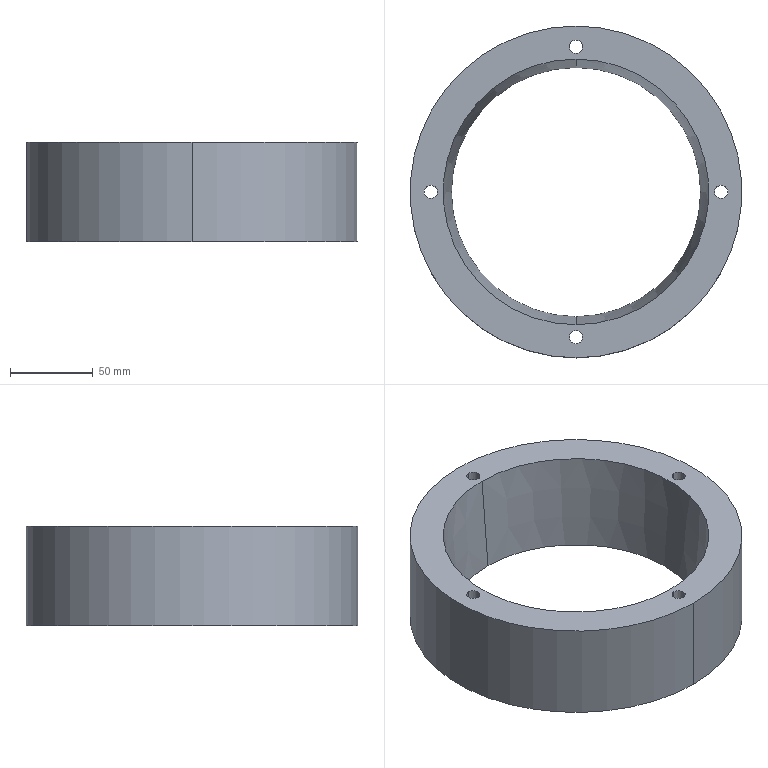Component | SolidWorks | DieStressRing-1 | 1 solid | 26 faces | box 200 x 200 x 60 mm | volume 718694 mm3 | cylinder 18 | plane 6 | cone 2 | commonest cylinder face diameters 16.5 x8 8 x8 200 x2
STEP:
#1=COLOUR_RGB('',0.7922,0.8196,0.9333);
#2=FILL_AREA_STYLE_COLOUR('',#1);
#3=FILL_AREA_STYLE('',(#2));
#4=SURFACE_STYLE_FILL_AREA(#3);
#5=SURFACE_SIDE_STYLE('',(#4));
#6=SURFACE_STYLE_USAGE(.BOTH.,#5);
#7=PRESENTATION_STYLE_ASSIGNMENT((#6));
#8=CARTESIAN_POINT('',(0.,-3.77,-3.071));
#9=VERTEX_POINT('',#8);
#10=CARTESIAN_POINT('',(0.,-3.12,-3.071));
#11=VERTEX_POINT('',#10);
#12=CARTESIAN_POINT('',(0.,-3.445,-3.071));
#13=DIRECTION('',(0.,0.,-1.));
#14=DIRECTION('',(-0.,1.,0.));
#15=AXIS2_PLACEMENT_3D('',#12,#13,#14);
#16=CIRCLE('',#15,0.3248);
#17=EDGE_CURVE('',#9,#11,#16,.T.);
#18=ORIENTED_EDGE('',*,*,#17,.F.);
#19=CARTESIAN_POINT('',(0.,-3.77,-4.252));
#20=VERTEX_POINT('',#19);
#21=CARTESIAN_POINT('',(0.,-3.77,-3.071));
#22=DIRECTION('',(0.,0.,-1.));
#23=VECTOR('',#22,39.37);
#24=LINE('',#21,#23);
#25=EDGE_CURVE('',#9,#20,#24,.T.);
#26=ORIENTED_EDGE('',*,*,#25,.T.);
#27=CARTESIAN_POINT('',(0.,-3.12,-4.252));
#28=VERTEX_POINT('',#27);
#29=CARTESIAN_POINT('',(0.,-3.445,-4.252));
#30=DIRECTION('',(0.,0.,-1.));
#31=DIRECTION('',(-0.,1.,0.));
#32=AXIS2_PLACEMENT_3D('',#29,#30,#31);
#33=CIRCLE('',#32,0.3248);
#34=EDGE_CURVE('',#20,#28,#33,.T.);
#35=ORIENTED_EDGE('',*,*,#34,.T.);
#36=CARTESIAN_POINT('',(0.,-3.12,-3.071));
#37=DIRECTION('',(0.,0.,-1.));
#38=VECTOR('',#37,39.37);
#39=LINE('',#36,#38);
#40=EDGE_CURVE('',#11,#28,#39,.T.);
#41=ORIENTED_EDGE('',*,*,#40,.F.);
#42=EDGE_LOOP('',(#18,#26,#35,#41));
#43=FACE_OUTER_BOUND('',#42,.T.);
#44=CARTESIAN_POINT('',(0.,-3.445,-3.071));
#45=DIRECTION('',(0.,0.,-1.));
#46=DIRECTION('',(-0.,1.,0.));
#47=AXIS2_PLACEMENT_3D('',#44,#45,#46);
#48=CYLINDRICAL_SURFACE('',#47,0.3248);
#49=ADVANCED_FACE('',(#43),#48,.F.);
#50=CARTESIAN_POINT('',(3.445,-0.3248,-3.071));
#51=VERTEX_POINT('',#50);
#52=CARTESIAN_POINT('',(3.445,0.3248,-3.071));
#53=VERTEX_POINT('',#52);
#54=CARTESIAN_POINT('',(3.445,-0.,-3.071));
#55=DIRECTION('',(0.,0.,-1.));
#56=DIRECTION('',(0.,1.,0.));
#57=AXIS2_PLACEMENT_3D('',#54,#55,#56);
#58=CIRCLE('',#57,0.3248);
#59=EDGE_CURVE('',#51,#53,#58,.T.);
#60=ORIENTED_EDGE('',*,*,#59,.F.);
#61=CARTESIAN_POINT('',(3.445,-0.3248,-4.252));
#62=VERTEX_POINT('',#61);
#63=CARTESIAN_POINT('',(3.445,-0.3248,-3.071));
#64=DIRECTION('',(0.,0.,-1.));
#65=VECTOR('',#64,39.37);
#66=LINE('',#63,#65);
#67=EDGE_CURVE('',#51,#62,#66,.T.);
#68=ORIENTED_EDGE('',*,*,#67,.T.);
#69=CARTESIAN_POINT('',(3.445,0.3248,-4.252));
#70=VERTEX_POINT('',#69);
#71=CARTESIAN_POINT('',(3.445,-0.,-4.252));
#72=DIRECTION('',(0.,0.,-1.));
#73=DIRECTION('',(0.,1.,0.));
#74=AXIS2_PLACEMENT_3D('',#71,#72,#73);
#75=CIRCLE('',#74,0.3248);
#76=EDGE_CURVE('',#62,#70,#75,.T.);
#77=ORIENTED_EDGE('',*,*,#76,.T.);
#78=CARTESIAN_POINT('',(3.445,0.3248,-3.071));
#79=DIRECTION('',(0.,0.,-1.));
#80=VECTOR('',#79,39.37);
#81=LINE('',#78,#80);
#82=EDGE_CURVE('',#53,#70,#81,.T.);
#83=ORIENTED_EDGE('',*,*,#82,.F.);
#84=EDGE_LOOP('',(#60,#68,#77,#83));
#85=FACE_OUTER_BOUND('',#84,.T.);
#86=CARTESIAN_POINT('',(3.445,-0.,-3.071));
#87=DIRECTION('',(0.,0.,-1.));
#88=DIRECTION('',(0.,1.,0.));
#89=AXIS2_PLACEMENT_3D('',#86,#87,#88);
#90=CYLINDRICAL_SURFACE('',#89,0.3248);
#91=ADVANCED_FACE('',(#85),#90,.F.);
#92=CARTESIAN_POINT('',(0.,3.12,-3.071));
#93=VERTEX_POINT('',#92);
#94=CARTESIAN_POINT('',(0.,3.77,-3.071));
#95=VERTEX_POINT('',#94);
#96=CARTESIAN_POINT('',(0.,3.445,-3.071));
#97=DIRECTION('',(0.,0.,-1.));
#98=DIRECTION('',(-0.,1.,0.));
#99=AXIS2_PLACEMENT_3D('',#96,#97,#98);
#100=CIRCLE('',#99,0.3248);
#101=EDGE_CURVE('',#93,#95,#100,.T.);
#102=ORIENTED_EDGE('',*,*,#101,.F.);
#103=CARTESIAN_POINT('',(0.,3.12,-4.252));
#104=VERTEX_POINT('',#103);
#105=CARTESIAN_POINT('',(0.,3.12,-3.071));
#106=DIRECTION('',(0.,0.,-1.));
#107=VECTOR('',#106,39.37);
#108=LINE('',#105,#107);
#109=EDGE_CURVE('',#93,#104,#108,.T.);
#110=ORIENTED_EDGE('',*,*,#109,.T.);
#111=CARTESIAN_POINT('',(0.,3.77,-4.252));
#112=VERTEX_POINT('',#111);
#113=CARTESIAN_POINT('',(0.,3.445,-4.252));
#114=DIRECTION('',(0.,0.,-1.));
#115=DIRECTION('',(-0.,1.,0.));
#116=AXIS2_PLACEMENT_3D('',#113,#114,#115);
#117=CIRCLE('',#116,0.3248);
#118=EDGE_CURVE('',#104,#112,#117,.T.);
#119=ORIENTED_EDGE('',*,*,#118,.T.);
#120=CARTESIAN_POINT('',(0.,3.77,-3.071));
#121=DIRECTION('',(0.,0.,-1.));
#122=VECTOR('',#121,39.37);
#123=LINE('',#120,#122);
#124=EDGE_CURVE('',#95,#112,#123,.T.);
#125=ORIENTED_EDGE('',*,*,#124,.F.);
#126=EDGE_LOOP('',(#102,#110,#119,#125));
#127=FACE_OUTER_BOUND('',#126,.T.);
#128=CARTESIAN_POINT('',(0.,3.445,-3.071));
#129=DIRECTION('',(0.,0.,-1.));
#130=DIRECTION('',(-0.,1.,0.));
#131=AXIS2_PLACEMENT_3D('',#128,#129,#130);
#132=CYLINDRICAL_SURFACE('',#131,0.3248);
#133=ADVANCED_FACE('',(#127),#132,.F.);
#134=CARTESIAN_POINT('',(-3.445,-0.3248,-3.071));
#135=VERTEX_POINT('',#134);
#136=CARTESIAN_POINT('',(-3.445,0.3248,-3.071));
#137=VERTEX_POINT('',#136);
#138=CARTESIAN_POINT('',(-3.445,-0.,-3.071));
#139=DIRECTION('',(0.,0.,-1.));
#140=DIRECTION('',(0.,1.,0.));
#141=AXIS2_PLACEMENT_3D('',#138,#139,#140);
#142=CIRCLE('',#141,0.3248);
#143=EDGE_CURVE('',#135,#137,#142,.T.);
#144=ORIENTED_EDGE('',*,*,#143,.F.);
#145=CARTESIAN_POINT('',(-3.445,-0.3248,-4.252));
#146=VERTEX_POINT('',#145);
#147=CARTESIAN_POINT('',(-3.445,-0.3248,-3.071));
#148=DIRECTION('',(0.,0.,-1.));
#149=VECTOR('',#148,39.37);
#150=LINE('',#147,#149);
#151=EDGE_CURVE('',#135,#146,#150,.T.);
#152=ORIENTED_EDGE('',*,*,#151,.T.);
#153=CARTESIAN_POINT('',(-3.445,0.3248,-4.252));
#154=VERTEX_POINT('',#153);
#155=CARTESIAN_POINT('',(-3.445,-0.,-4.252));
#156=DIRECTION('',(0.,0.,-1.));
#157=DIRECTION('',(0.,1.,0.));
#158=AXIS2_PLACEMENT_3D('',#155,#156,#157);
#159=CIRCLE('',#158,0.3248);
#160=EDGE_CURVE('',#146,#154,#159,.T.);
#161=ORIENTED_EDGE('',*,*,#160,.T.);
#162=CARTESIAN_POINT('',(-3.445,0.3248,-3.071));
#163=DIRECTION('',(0.,0.,-1.));
#164=VECTOR('',#163,39.37);
#165=LINE('',#162,#164);
#166=EDGE_CURVE('',#137,#154,#165,.T.);
#167=ORIENTED_EDGE('',*,*,#166,.F.);
#168=EDGE_LOOP('',(#144,#152,#161,#167));
#169=FACE_OUTER_BOUND('',#168,.T.);
#170=CARTESIAN_POINT('',(-3.445,-0.,-3.071));
#171=DIRECTION('',(0.,0.,-1.));
#172=DIRECTION('',(0.,1.,0.));
#173=AXIS2_PLACEMENT_3D('',#170,#171,#172);
#174=CYLINDRICAL_SURFACE('',#173,0.3248);
#175=ADVANCED_FACE('',(#169),#174,.F.);
#176=CARTESIAN_POINT('',(0.,-3.937,-4.252));
#177=VERTEX_POINT('',#176);
#178=CARTESIAN_POINT('',(-0.,3.937,-4.252));
#179=VERTEX_POINT('',#178);
#180=CARTESIAN_POINT('',(0.,0.,-4.252));
#181=DIRECTION('',(0.,0.,1.));
#182=DIRECTION('',(0.,-1.,0.));
#183=AXIS2_PLACEMENT_3D('',#180,#181,#182);
#184=CIRCLE('',#183,3.937);
#185=EDGE_CURVE('',#177,#179,#184,.T.);
#186=ORIENTED_EDGE('',*,*,#185,.T.);
#187=CARTESIAN_POINT('',(-0.,3.937,-1.89));
#188=VERTEX_POINT('',#187);
#189=CARTESIAN_POINT('',(-0.,3.937,-1.89));
#190=DIRECTION('',(0.,0.,1.));
#191=VECTOR('',#190,39.37);
#192=LINE('',#189,#191);
#193=EDGE_CURVE('',#179,#188,#192,.T.);
#194=ORIENTED_EDGE('',*,*,#193,.T.);
#195=CARTESIAN_POINT('',(0.,-3.937,-1.89));
#196=VERTEX_POINT('',#195);
#197=CARTESIAN_POINT('',(0.,0.,-1.89));
#198=DIRECTION('',(0.,0.,1.));
#199=DIRECTION('',(0.,-1.,0.));
#200=AXIS2_PLACEMENT_3D('',#197,#198,#199);
#201=CIRCLE('',#200,3.937);
#202=EDGE_CURVE('',#196,#188,#201,.T.);
#203=ORIENTED_EDGE('',*,*,#202,.F.);
#204=CARTESIAN_POINT('',(0.,-3.937,-1.89));
#205=DIRECTION('',(0.,0.,1.));
#206=VECTOR('',#205,39.37);
#207=LINE('',#204,#206);
#208=EDGE_CURVE('',#177,#196,#207,.T.);
#209=ORIENTED_EDGE('',*,*,#208,.F.);
#210=EDGE_LOOP('',(#186,#194,#203,#209));
#211=FACE_OUTER_BOUND('',#210,.T.);
#212=CARTESIAN_POINT('',(0.,0.,-1.89));
#213=DIRECTION('',(0.,0.,1.));
#214=DIRECTION('',(0.,-1.,0.));
#215=AXIS2_PLACEMENT_3D('',#212,#213,#214);
#216=CYLINDRICAL_SURFACE('',#215,3.937);
#217=ADVANCED_FACE('',(#211),#216,.T.);
#218=CARTESIAN_POINT('',(-3.445,0.1575,-3.071));
#219=VERTEX_POINT('',#218);
#220=CARTESIAN_POINT('',(-3.445,-0.1575,-3.071));
#221=VERTEX_POINT('',#220);
#222=CARTESIAN_POINT('',(-3.445,-0.,-3.071));
#223=DIRECTION('',(0.,0.,1.));
#224=DIRECTION('',(0.,1.,0.));
#225=AXIS2_PLACEMENT_3D('',#222,#223,#224);
#226=CIRCLE('',#225,0.1575);
#227=EDGE_CURVE('',#219,#221,#226,.T.);
#228=ORIENTED_EDGE('',*,*,#227,.F.);
#229=CARTESIAN_POINT('',(-3.445,0.1575,-1.89));
#230=VERTEX_POINT('',#229);
#231=CARTESIAN_POINT('',(-3.445,0.1575,-2.48));
#232=DIRECTION('',(0.,0.,1.));
#233=VECTOR('',#232,39.37);
#234=LINE('',#231,#233);
#235=EDGE_CURVE('',#219,#230,#234,.T.);
#236=ORIENTED_EDGE('',*,*,#235,.T.);
#237=CARTESIAN_POINT('',(-3.445,-0.1575,-1.89));
#238=VERTEX_POINT('',#237);
#239=CARTESIAN_POINT('',(-3.445,-0.,-1.89));
#240=DIRECTION('',(0.,0.,1.));
#241=DIRECTION('',(0.,-1.,0.));
#242=AXIS2_PLACEMENT_3D('',#239,#240,#241);
#243=CIRCLE('',#242,0.1575);
#244=EDGE_CURVE('',#230,#238,#243,.T.);
#245=ORIENTED_EDGE('',*,*,#244,.T.);
#246=CARTESIAN_POINT('',(-3.445,-0.1575,-2.48));
#247=DIRECTION('',(0.,0.,1.));
#248=VECTOR('',#247,39.37);
#249=LINE('',#246,#248);
#250=EDGE_CURVE('',#221,#238,#249,.T.);
#251=ORIENTED_EDGE('',*,*,#250,.F.);
#252=EDGE_LOOP('',(#228,#236,#245,#251));
#253=FACE_OUTER_BOUND('',#252,.T.);
#254=CARTESIAN_POINT('',(-3.445,-0.,-2.48));
#255=DIRECTION('',(0.,0.,1.));
#256=DIRECTION('',(0.,-1.,0.));
#257=AXIS2_PLACEMENT_3D('',#254,#255,#256);
#258=CYLINDRICAL_SURFACE('',#257,0.1575);
#259=ADVANCED_FACE('',(#253),#258,.F.);
#260=CARTESIAN_POINT('',(0.,3.602,-3.071));
#261=VERTEX_POINT('',#260);
#262=CARTESIAN_POINT('',(0.,3.287,-3.071));
#263=VERTEX_POINT('',#262);
#264=CARTESIAN_POINT('',(0.,3.445,-3.071));
#265=DIRECTION('',(0.,0.,1.));
#266=DIRECTION('',(-0.,1.,0.));
#267=AXIS2_PLACEMENT_3D('',#264,#265,#266);
#268=CIRCLE('',#267,0.1575);
#269=EDGE_CURVE('',#261,#263,#268,.T.);
#270=ORIENTED_EDGE('',*,*,#269,.F.);
#271=CARTESIAN_POINT('',(0.,3.602,-1.89));
#272=VERTEX_POINT('',#271);
#273=CARTESIAN_POINT('',(0.,3.602,-2.48));
#274=DIRECTION('',(0.,0.,1.));
#275=VECTOR('',#274,39.37);
#276=LINE('',#273,#275);
#277=EDGE_CURVE('',#261,#272,#276,.T.);
#278=ORIENTED_EDGE('',*,*,#277,.T.);
#279=CARTESIAN_POINT('',(0.,3.287,-1.89));
#280=VERTEX_POINT('',#279);
#281=CARTESIAN_POINT('',(0.,3.445,-1.89));
#282=DIRECTION('',(0.,0.,1.));
#283=DIRECTION('',(0.,-1.,0.));
#284=AXIS2_PLACEMENT_3D('',#281,#282,#283);
#285=CIRCLE('',#284,0.1575);
#286=EDGE_CURVE('',#272,#280,#285,.T.);
#287=ORIENTED_EDGE('',*,*,#286,.T.);
#288=CARTESIAN_POINT('',(0.,3.287,-2.48));
#289=DIRECTION('',(0.,0.,1.));
#290=VECTOR('',#289,39.37);
#291=LINE('',#288,#290);
#292=EDGE_CURVE('',#263,#280,#291,.T.);
#293=ORIENTED_EDGE('',*,*,#292,.F.);
#294=EDGE_LOOP('',(#270,#278,#287,#293));
#295=FACE_OUTER_BOUND('',#294,.T.);
#296=CARTESIAN_POINT('',(0.,3.445,-2.48));
#297=DIRECTION('',(0.,0.,1.));
#298=DIRECTION('',(0.,-1.,0.));
#299=AXIS2_PLACEMENT_3D('',#296,#297,#298);
#300=CYLINDRICAL_SURFACE('',#299,0.1575);
#301=ADVANCED_FACE('',(#295),#300,.F.);
#302=CARTESIAN_POINT('',(3.445,0.1575,-3.071));
#303=VERTEX_POINT('',#302);
#304=CARTESIAN_POINT('',(3.445,-0.1575,-3.071));
#305=VERTEX_POINT('',#304);
#306=CARTESIAN_POINT('',(3.445,-0.,-3.071));
#307=DIRECTION('',(0.,0.,1.));
#308=DIRECTION('',(0.,1.,0.));
#309=AXIS2_PLACEMENT_3D('',#306,#307,#308);
#310=CIRCLE('',#309,0.1575);
#311=EDGE_CURVE('',#303,#305,#310,.T.);
#312=ORIENTED_EDGE('',*,*,#311,.F.);
#313=CARTESIAN_POINT('',(3.445,0.1575,-1.89));
#314=VERTEX_POINT('',#313);
#315=CARTESIAN_POINT('',(3.445,0.1575,-2.48));
#316=DIRECTION('',(0.,0.,1.));
#317=VECTOR('',#316,39.37);
#318=LINE('',#315,#317);
#319=EDGE_CURVE('',#303,#314,#318,.T.);
#320=ORIENTED_EDGE('',*,*,#319,.T.);
#321=CARTESIAN_POINT('',(3.445,-0.1575,-1.89));
#322=VERTEX_POINT('',#321);
#323=CARTESIAN_POINT('',(3.445,-0.,-1.89));
#324=DIRECTION('',(0.,0.,1.));
#325=DIRECTION('',(0.,-1.,0.));
#326=AXIS2_PLACEMENT_3D('',#323,#324,#325);
#327=CIRCLE('',#326,0.1575);
#328=EDGE_CURVE('',#314,#322,#327,.T.);
#329=ORIENTED_EDGE('',*,*,#328,.T.);
#330=CARTESIAN_POINT('',(3.445,-0.1575,-2.48));
#331=DIRECTION('',(0.,0.,1.));
#332=VECTOR('',#331,39.37);
#333=LINE('',#330,#332);
#334=EDGE_CURVE('',#305,#322,#333,.T.);
#335=ORIENTED_EDGE('',*,*,#334,.F.);
#336=EDGE_LOOP('',(#312,#320,#329,#335));
#337=FACE_OUTER_BOUND('',#336,.T.);
#338=CARTESIAN_POINT('',(3.445,-0.,-2.48));
#339=DIRECTION('',(0.,0.,1.));
#340=DIRECTION('',(0.,-1.,0.));
#341=AXIS2_PLACEMENT_3D('',#338,#339,#340);
#342=CYLINDRICAL_SURFACE('',#341,0.1575);
#343=ADVANCED_FACE('',(#337),#342,.F.);
#344=CARTESIAN_POINT('',(-0.,-3.287,-3.071));
#345=VERTEX_POINT('',#344);
#346=CARTESIAN_POINT('',(0.,-3.602,-3.071));
#347=VERTEX_POINT('',#346);
#348=CARTESIAN_POINT('',(-0.,-3.445,-3.071));
#349=DIRECTION('',(0.,0.,1.));
#350=DIRECTION('',(-0.,1.,0.));
#351=AXIS2_PLACEMENT_3D('',#348,#349,#350);
#352=CIRCLE('',#351,0.1575);
#353=EDGE_CURVE('',#345,#347,#352,.T.);
#354=ORIENTED_EDGE('',*,*,#353,.F.);
#355=CARTESIAN_POINT('',(-0.,-3.287,-1.89));
#356=VERTEX_POINT('',#355);
#357=CARTESIAN_POINT('',(-0.,-3.287,-2.48));
#358=DIRECTION('',(0.,0.,1.));
#359=VECTOR('',#358,39.37);
#360=LINE('',#357,#359);
#361=EDGE_CURVE('',#345,#356,#360,.T.);
#362=ORIENTED_EDGE('',*,*,#361,.T.);
#363=CARTESIAN_POINT('',(0.,-3.602,-1.89));
#364=VERTEX_POINT('',#363);
#365=CARTESIAN_POINT('',(-0.,-3.445,-1.89));
#366=DIRECTION('',(0.,0.,1.));
#367=DIRECTION('',(0.,-1.,0.));
#368=AXIS2_PLACEMENT_3D('',#365,#366,#367);
#369=CIRCLE('',#368,0.1575);
#370=EDGE_CURVE('',#356,#364,#369,.T.);
#371=ORIENTED_EDGE('',*,*,#370,.T.);
#372=CARTESIAN_POINT('',(0.,-3.602,-2.48));
#373=DIRECTION('',(0.,0.,1.));
#374=VECTOR('',#373,39.37);
#375=LINE('',#372,#374);
#376=EDGE_CURVE('',#347,#364,#375,.T.);
#377=ORIENTED_EDGE('',*,*,#376,.F.);
#378=EDGE_LOOP('',(#354,#362,#371,#377));
#379=FACE_OUTER_BOUND('',#378,.T.);
#380=CARTESIAN_POINT('',(-0.,-3.445,-2.48));
#381=DIRECTION('',(0.,0.,1.));
#382=DIRECTION('',(0.,-1.,0.));
#383=AXIS2_PLACEMENT_3D('',#380,#381,#382);
#384=CYLINDRICAL_SURFACE('',#383,0.1575);
#385=ADVANCED_FACE('',(#379),#384,.F.);
#386=CARTESIAN_POINT('',(0.,-2.955,-4.252));
#387=VERTEX_POINT('',#386);
#388=CARTESIAN_POINT('',(-0.,2.955,-4.252));
#389=VERTEX_POINT('',#388);
#390=CARTESIAN_POINT('',(0.,0.,-4.252));
#391=DIRECTION('',(0.,0.,-1.));
#392=DIRECTION('',(-0.,1.,0.));
#393=AXIS2_PLACEMENT_3D('',#390,#391,#392);
#394=CIRCLE('',#393,2.955);
#395=EDGE_CURVE('',#387,#389,#394,.T.);
#396=ORIENTED_EDGE('',*,*,#395,.T.);
#397=CARTESIAN_POINT('',(-0.,3.152,-1.89));
#398=VERTEX_POINT('',#397);
#399=CARTESIAN_POINT('',(-0.,3.147,-1.955));
#400=DIRECTION('',(-0.,0.08305,0.9965));
#401=VECTOR('',#400,39.37);
#402=LINE('',#399,#401);
#403=EDGE_CURVE('',#389,#398,#402,.T.);
#404=ORIENTED_EDGE('',*,*,#403,.T.);
#405=CARTESIAN_POINT('',(0.,-3.152,-1.89));
#406=VERTEX_POINT('',#405);
#407=CARTESIAN_POINT('',(0.,0.,-1.89));
#408=DIRECTION('',(0.,0.,1.));
#409=DIRECTION('',(0.,-1.,0.));
#410=AXIS2_PLACEMENT_3D('',#407,#408,#409);
#411=CIRCLE('',#410,3.152);
#412=EDGE_CURVE('',#398,#406,#411,.T.);
#413=ORIENTED_EDGE('',*,*,#412,.T.);
#414=CARTESIAN_POINT('',(0.,-3.147,-1.955));
#415=DIRECTION('',(0.,-0.08305,0.9965));
#416=VECTOR('',#415,39.37);
#417=LINE('',#414,#416);
#418=EDGE_CURVE('',#387,#406,#417,.T.);
#419=ORIENTED_EDGE('',*,*,#418,.F.);
#420=EDGE_LOOP('',(#396,#404,#413,#419));
#421=FACE_OUTER_BOUND('',#420,.T.);
#422=CARTESIAN_POINT('',(0.,0.,-1.955));
#423=DIRECTION('',(0.,0.,1.));
#424=DIRECTION('',(0.,-1.,0.));
#425=AXIS2_PLACEMENT_3D('',#422,#423,#424);
#426=CONICAL_SURFACE('',#425,3.147,0.08314);
#427=ADVANCED_FACE('',(#421),#426,.F.);
#428=ORIENTED_EDGE('',*,*,#403,.F.);
#429=CARTESIAN_POINT('',(0.,0.,-4.252));
#430=DIRECTION('',(0.,0.,-1.));
#431=DIRECTION('',(-0.,1.,0.));
#432=AXIS2_PLACEMENT_3D('',#429,#430,#431);
#433=CIRCLE('',#432,2.955);
#434=EDGE_CURVE('',#389,#387,#433,.T.);
#435=ORIENTED_EDGE('',*,*,#434,.T.);
#436=ORIENTED_EDGE('',*,*,#418,.T.);
#437=CARTESIAN_POINT('',(0.,0.,-1.89));
#438=DIRECTION('',(0.,0.,1.));
#439=DIRECTION('',(0.,-1.,0.));
#440=AXIS2_PLACEMENT_3D('',#437,#438,#439);
#441=CIRCLE('',#440,3.152);
#442=EDGE_CURVE('',#406,#398,#441,.T.);
#443=ORIENTED_EDGE('',*,*,#442,.T.);
#444=EDGE_LOOP('',(#428,#435,#436,#443));
#445=FACE_OUTER_BOUND('',#444,.T.);
#446=CARTESIAN_POINT('',(0.,0.,-1.955));
#447=DIRECTION('',(0.,0.,1.));
#448=DIRECTION('',(0.,-1.,0.));
#449=AXIS2_PLACEMENT_3D('',#446,#447,#448);
#450=CONICAL_SURFACE('',#449,3.147,0.08314);
#451=ADVANCED_FACE('',(#445),#450,.F.);
#452=ORIENTED_EDGE('',*,*,#361,.F.);
#453=CARTESIAN_POINT('',(-0.,-3.445,-3.071));
#454=DIRECTION('',(0.,0.,1.));
#455=DIRECTION('',(-0.,1.,0.));
#456=AXIS2_PLACEMENT_3D('',#453,#454,#455);
#457=CIRCLE('',#456,0.1575);
#458=EDGE_CURVE('',#347,#345,#457,.T.);
#459=ORIENTED_EDGE('',*,*,#458,.F.);
#460=ORIENTED_EDGE('',*,*,#376,.T.);
#461=CARTESIAN_POINT('',(-0.,-3.445,-1.89));
#462=DIRECTION('',(0.,0.,1.));
#463=DIRECTION('',(0.,-1.,0.));
#464=AXIS2_PLACEMENT_3D('',#461,#462,#463);
#465=CIRCLE('',#464,0.1575);
#466=EDGE_CURVE('',#364,#356,#465,.T.);
#467=ORIENTED_EDGE('',*,*,#466,.T.);
#468=EDGE_LOOP('',(#452,#459,#460,#467));
#469=FACE_OUTER_BOUND('',#468,.T.);
#470=CARTESIAN_POINT('',(-0.,-3.445,-2.48));
#471=DIRECTION('',(0.,0.,1.));
#472=DIRECTION('',(0.,-1.,0.));
#473=AXIS2_PLACEMENT_3D('',#470,#471,#472);
#474=CYLINDRICAL_SURFACE('',#473,0.1575);
#475=ADVANCED_FACE('',(#469),#474,.F.);
#476=ORIENTED_EDGE('',*,*,#319,.F.);
#477=CARTESIAN_POINT('',(3.445,-0.,-3.071));
#478=DIRECTION('',(0.,0.,1.));
#479=DIRECTION('',(0.,1.,0.));
#480=AXIS2_PLACEMENT_3D('',#477,#478,#479);
#481=CIRCLE('',#480,0.1575);
#482=EDGE_CURVE('',#305,#303,#481,.T.);
#483=ORIENTED_EDGE('',*,*,#482,.F.);
#484=ORIENTED_EDGE('',*,*,#334,.T.);
#485=CARTESIAN_POINT('',(3.445,-0.,-1.89));
#486=DIRECTION('',(0.,0.,1.));
#487=DIRECTION('',(0.,-1.,0.));
#488=AXIS2_PLACEMENT_3D('',#485,#486,#487);
#489=CIRCLE('',#488,0.1575);
#490=EDGE_CURVE('',#322,#314,#489,.T.);
#491=ORIENTED_EDGE('',*,*,#490,.T.);
#492=EDGE_LOOP('',(#476,#483,#484,#491));
#493=FACE_OUTER_BOUND('',#492,.T.);
#494=CARTESIAN_POINT('',(3.445,-0.,-2.48));
#495=DIRECTION('',(0.,0.,1.));
#496=DIRECTION('',(0.,-1.,0.));
#497=AXIS2_PLACEMENT_3D('',#494,#495,#496);
#498=CYLINDRICAL_SURFACE('',#497,0.1575);
#499=ADVANCED_FACE('',(#493),#498,.F.);
#500=ORIENTED_EDGE('',*,*,#277,.F.);
#501=CARTESIAN_POINT('',(0.,3.445,-3.071));
#502=DIRECTION('',(0.,0.,1.));
#503=DIRECTION('',(-0.,1.,0.));
#504=AXIS2_PLACEMENT_3D('',#501,#502,#503);
#505=CIRCLE('',#504,0.1575);
#506=EDGE_CURVE('',#263,#261,#505,.T.);
#507=ORIENTED_EDGE('',*,*,#506,.F.);
#508=ORIENTED_EDGE('',*,*,#292,.T.);
#509=CARTESIAN_POINT('',(0.,3.445,-1.89));
#510=DIRECTION('',(0.,0.,1.));
#511=DIRECTION('',(0.,-1.,0.));
#512=AXIS2_PLACEMENT_3D('',#509,#510,#511);
#513=CIRCLE('',#512,0.1575);
#514=EDGE_CURVE('',#280,#272,#513,.T.);
#515=ORIENTED_EDGE('',*,*,#514,.T.);
#516=EDGE_LOOP('',(#500,#507,#508,#515));
#517=FACE_OUTER_BOUND('',#516,.T.);
#518=CARTESIAN_POINT('',(0.,3.445,-2.48));
#519=DIRECTION('',(0.,0.,1.));
#520=DIRECTION('',(0.,-1.,0.));
#521=AXIS2_PLACEMENT_3D('',#518,#519,#520);
#522=CYLINDRICAL_SURFACE('',#521,0.1575);
#523=ADVANCED_FACE('',(#517),#522,.F.);
#524=ORIENTED_EDGE('',*,*,#235,.F.);
#525=CARTESIAN_POINT('',(-3.445,-0.,-3.071));
#526=DIRECTION('',(0.,0.,1.));
#527=DIRECTION('',(0.,1.,0.));
#528=AXIS2_PLACEMENT_3D('',#525,#526,#527);
#529=CIRCLE('',#528,0.1575);
#530=EDGE_CURVE('',#221,#219,#529,.T.);
#531=ORIENTED_EDGE('',*,*,#530,.F.);
#532=ORIENTED_EDGE('',*,*,#250,.T.);
#533=CARTESIAN_POINT('',(-3.445,-0.,-1.89));
#534=DIRECTION('',(0.,0.,1.));
#535=DIRECTION('',(0.,-1.,0.));
#536=AXIS2_PLACEMENT_3D('',#533,#534,#535);
#537=CIRCLE('',#536,0.1575);
#538=EDGE_CURVE('',#238,#230,#537,.T.);
#539=ORIENTED_EDGE('',*,*,#538,.T.);
#540=EDGE_LOOP('',(#524,#531,#532,#539));
#541=FACE_OUTER_BOUND('',#540,.T.);
#542=CARTESIAN_POINT('',(-3.445,-0.,-2.48));
#543=DIRECTION('',(0.,0.,1.));
#544=DIRECTION('',(0.,-1.,0.));
#545=AXIS2_PLACEMENT_3D('',#542,#543,#544);
#546=CYLINDRICAL_SURFACE('',#545,0.1575);
#547=ADVANCED_FACE('',(#541),#546,.F.);
#548=CARTESIAN_POINT('',(-3.445,-0.,-4.252));
#549=DIRECTION('',(0.,0.,-1.));
#550=DIRECTION('',(0.,1.,0.));
#551=AXIS2_PLACEMENT_3D('',#548,#549,#550);
#552=CIRCLE('',#551,0.3248);
#553=EDGE_CURVE('',#154,#146,#552,.T.);
#554=ORIENTED_EDGE('',*,*,#553,.F.);
#555=ORIENTED_EDGE('',*,*,#160,.F.);
#556=EDGE_LOOP('',(#554,#555));
#557=FACE_BOUND('',#556,.T.);
#558=CARTESIAN_POINT('',(0.,-3.445,-4.252));
#559=DIRECTION('',(0.,0.,-1.));
#560=DIRECTION('',(-0.,1.,0.));
#561=AXIS2_PLACEMENT_3D('',#558,#559,#560);
#562=CIRCLE('',#561,0.3248);
#563=EDGE_CURVE('',#28,#20,#562,.T.);
#564=ORIENTED_EDGE('',*,*,#563,.F.);
#565=ORIENTED_EDGE('',*,*,#34,.F.);
#566=EDGE_LOOP('',(#564,#565));
#567=FACE_BOUND('',#566,.T.);
#568=CARTESIAN_POINT('',(3.445,-0.,-4.252));
#569=DIRECTION('',(0.,0.,-1.));
#570=DIRECTION('',(0.,1.,0.));
#571=AXIS2_PLACEMENT_3D('',#568,#569,#570);
#572=CIRCLE('',#571,0.3248);
#573=EDGE_CURVE('',#70,#62,#572,.T.);
#574=ORIENTED_EDGE('',*,*,#573,.F.);
#575=ORIENTED_EDGE('',*,*,#76,.F.);
#576=EDGE_LOOP('',(#574,#575));
#577=FACE_BOUND('',#576,.T.);
#578=CARTESIAN_POINT('',(0.,3.445,-4.252));
#579=DIRECTION('',(0.,0.,-1.));
#580=DIRECTION('',(-0.,1.,0.));
#581=AXIS2_PLACEMENT_3D('',#578,#579,#580);
#582=CIRCLE('',#581,0.3248);
#583=EDGE_CURVE('',#112,#104,#582,.T.);
#584=ORIENTED_EDGE('',*,*,#583,.F.);
#585=ORIENTED_EDGE('',*,*,#118,.F.);
#586=EDGE_LOOP('',(#584,#585));
#587=FACE_BOUND('',#586,.T.);
#588=ORIENTED_EDGE('',*,*,#395,.F.);
#589=ORIENTED_EDGE('',*,*,#434,.F.);
#590=EDGE_LOOP('',(#588,#589));
#591=FACE_BOUND('',#590,.T.);
#592=ORIENTED_EDGE('',*,*,#185,.F.);
#593=CARTESIAN_POINT('',(0.,0.,-4.252));
#594=DIRECTION('',(0.,0.,1.));
#595=DIRECTION('',(0.,-1.,0.));
#596=AXIS2_PLACEMENT_3D('',#593,#594,#595);
#597=CIRCLE('',#596,3.937);
#598=EDGE_CURVE('',#179,#177,#597,.T.);
#599=ORIENTED_EDGE('',*,*,#598,.F.);
#600=EDGE_LOOP('',(#592,#599));
#601=FACE_OUTER_BOUND('',#600,.T.);
#602=CARTESIAN_POINT('',(0.,0.,-4.252));
#603=DIRECTION('',(0.,0.,-1.));
#604=DIRECTION('',(-0.,1.,0.));
#605=AXIS2_PLACEMENT_3D('',#602,#603,#604);
#606=PLANE('',#605);
#607=ADVANCED_FACE('',(#557,#567,#577,#587,#591,#601),#606,.T.);
#608=ORIENTED_EDGE('',*,*,#193,.F.);
#609=ORIENTED_EDGE('',*,*,#598,.T.);
#610=ORIENTED_EDGE('',*,*,#208,.T.);
#611=CARTESIAN_POINT('',(0.,0.,-1.89));
#612=DIRECTION('',(0.,0.,1.));
#613=DIRECTION('',(0.,-1.,0.));
#614=AXIS2_PLACEMENT_3D('',#611,#612,#613);
#615=CIRCLE('',#614,3.937);
#616=EDGE_CURVE('',#188,#196,#615,.T.);
#617=ORIENTED_EDGE('',*,*,#616,.F.);
#618=EDGE_LOOP('',(#608,#609,#610,#617));
#619=FACE_OUTER_BOUND('',#618,.T.);
#620=CARTESIAN_POINT('',(0.,0.,-1.89));
#621=DIRECTION('',(0.,0.,1.));
#622=DIRECTION('',(0.,-1.,0.));
#623=AXIS2_PLACEMENT_3D('',#620,#621,#622);
#624=CYLINDRICAL_SURFACE('',#623,3.937);
#625=ADVANCED_FACE('',(#619),#624,.T.);
#626=ORIENTED_EDGE('',*,*,#538,.F.);
#627=ORIENTED_EDGE('',*,*,#244,.F.);
#628=EDGE_LOOP('',(#626,#627));
#629=FACE_BOUND('',#628,.T.);
#630=ORIENTED_EDGE('',*,*,#514,.F.);
#631=ORIENTED_EDGE('',*,*,#286,.F.);
#632=EDGE_LOOP('',(#630,#631));
#633=FACE_BOUND('',#632,.T.);
#634=ORIENTED_EDGE('',*,*,#490,.F.);
#635=ORIENTED_EDGE('',*,*,#328,.F.);
#636=EDGE_LOOP('',(#634,#635));
#637=FACE_BOUND('',#636,.T.);
#638=ORIENTED_EDGE('',*,*,#466,.F.);
#639=ORIENTED_EDGE('',*,*,#370,.F.);
#640=EDGE_LOOP('',(#638,#639));
#641=FACE_BOUND('',#640,.T.);
#642=ORIENTED_EDGE('',*,*,#202,.T.);
#643=ORIENTED_EDGE('',*,*,#616,.T.);
#644=EDGE_LOOP('',(#642,#643));
#645=FACE_OUTER_BOUND('',#644,.T.);
#646=ORIENTED_EDGE('',*,*,#442,.F.);
#647=ORIENTED_EDGE('',*,*,#412,.F.);
#648=EDGE_LOOP('',(#646,#647));
#649=FACE_BOUND('',#648,.T.);
#650=CARTESIAN_POINT('',(3.937,0.,-1.89));
#651=DIRECTION('',(0.,0.,1.));
#652=DIRECTION('',(0.,-1.,0.));
#653=AXIS2_PLACEMENT_3D('',#650,#651,#652);
#654=PLANE('',#653);
#655=ADVANCED_FACE('',(#629,#633,#637,#641,#645,#649),#654,.T.);
#656=CARTESIAN_POINT('',(-3.445,-0.,-3.071));
#657=DIRECTION('',(0.,0.,-1.));
#658=DIRECTION('',(0.,1.,0.));
#659=AXIS2_PLACEMENT_3D('',#656,#657,#658);
#660=CIRCLE('',#659,0.3248);
#661=EDGE_CURVE('',#137,#135,#660,.T.);
#662=ORIENTED_EDGE('',*,*,#661,.T.);
#663=ORIENTED_EDGE('',*,*,#143,.T.);
#664=EDGE_LOOP('',(#662,#663));
#665=FACE_OUTER_BOUND('',#664,.T.);
#666=ORIENTED_EDGE('',*,*,#530,.T.);
#667=ORIENTED_EDGE('',*,*,#227,.T.);
#668=EDGE_LOOP('',(#666,#667));
#669=FACE_BOUND('',#668,.T.);
#670=CARTESIAN_POINT('',(-3.445,-0.,-3.071));
#671=DIRECTION('',(0.,0.,-1.));
#672=DIRECTION('',(-0.,1.,0.));
#673=AXIS2_PLACEMENT_3D('',#670,#671,#672);
#674=PLANE('',#673);
#675=ADVANCED_FACE('',(#665,#669),#674,.T.);
#676=ORIENTED_EDGE('',*,*,#151,.F.);
#677=ORIENTED_EDGE('',*,*,#661,.F.);
#678=ORIENTED_EDGE('',*,*,#166,.T.);
#679=ORIENTED_EDGE('',*,*,#553,.T.);
#680=EDGE_LOOP('',(#676,#677,#678,#679));
#681=FACE_OUTER_BOUND('',#680,.T.);
#682=CARTESIAN_POINT('',(-3.445,-0.,-3.071));
#683=DIRECTION('',(0.,0.,-1.));
#684=DIRECTION('',(0.,1.,0.));
#685=AXIS2_PLACEMENT_3D('',#682,#683,#684);
#686=CYLINDRICAL_SURFACE('',#685,0.3248);
#687=ADVANCED_FACE('',(#681),#686,.F.);
#688=CARTESIAN_POINT('',(0.,3.445,-3.071));
#689=DIRECTION('',(0.,0.,-1.));
#690=DIRECTION('',(-0.,1.,0.));
#691=AXIS2_PLACEMENT_3D('',#688,#689,#690);
#692=CIRCLE('',#691,0.3248);
#693=EDGE_CURVE('',#95,#93,#692,.T.);
#694=ORIENTED_EDGE('',*,*,#693,.T.);
#695=ORIENTED_EDGE('',*,*,#101,.T.);
#696=EDGE_LOOP('',(#694,#695));
#697=FACE_OUTER_BOUND('',#696,.T.);
#698=ORIENTED_EDGE('',*,*,#506,.T.);
#699=ORIENTED_EDGE('',*,*,#269,.T.);
#700=EDGE_LOOP('',(#698,#699));
#701=FACE_BOUND('',#700,.T.);
#702=CARTESIAN_POINT('',(0.,3.445,-3.071));
#703=DIRECTION('',(0.,0.,-1.));
#704=DIRECTION('',(-0.,1.,0.));
#705=AXIS2_PLACEMENT_3D('',#702,#703,#704);
#706=PLANE('',#705);
#707=ADVANCED_FACE('',(#697,#701),#706,.T.);
#708=ORIENTED_EDGE('',*,*,#109,.F.);
#709=ORIENTED_EDGE('',*,*,#693,.F.);
#710=ORIENTED_EDGE('',*,*,#124,.T.);
#711=ORIENTED_EDGE('',*,*,#583,.T.);
#712=EDGE_LOOP('',(#708,#709,#710,#711));
#713=FACE_OUTER_BOUND('',#712,.T.);
#714=CARTESIAN_POINT('',(0.,3.445,-3.071));
#715=DIRECTION('',(0.,0.,-1.));
#716=DIRECTION('',(-0.,1.,0.));
#717=AXIS2_PLACEMENT_3D('',#714,#715,#716);
#718=CYLINDRICAL_SURFACE('',#717,0.3248);
#719=ADVANCED_FACE('',(#713),#718,.F.);
#720=CARTESIAN_POINT('',(3.445,-0.,-3.071));
#721=DIRECTION('',(0.,0.,-1.));
#722=DIRECTION('',(0.,1.,0.));
#723=AXIS2_PLACEMENT_3D('',#720,#721,#722);
#724=CIRCLE('',#723,0.3248);
#725=EDGE_CURVE('',#53,#51,#724,.T.);
#726=ORIENTED_EDGE('',*,*,#725,.T.);
#727=ORIENTED_EDGE('',*,*,#59,.T.);
#728=EDGE_LOOP('',(#726,#727));
#729=FACE_OUTER_BOUND('',#728,.T.);
#730=ORIENTED_EDGE('',*,*,#482,.T.);
#731=ORIENTED_EDGE('',*,*,#311,.T.);
#732=EDGE_LOOP('',(#730,#731));
#733=FACE_BOUND('',#732,.T.);
#734=CARTESIAN_POINT('',(3.445,-0.,-3.071));
#735=DIRECTION('',(0.,0.,-1.));
#736=DIRECTION('',(-0.,1.,0.));
#737=AXIS2_PLACEMENT_3D('',#734,#735,#736);
#738=PLANE('',#737);
#739=ADVANCED_FACE('',(#729,#733),#738,.T.);
#740=ORIENTED_EDGE('',*,*,#67,.F.);
#741=ORIENTED_EDGE('',*,*,#725,.F.);
#742=ORIENTED_EDGE('',*,*,#82,.T.);
#743=ORIENTED_EDGE('',*,*,#573,.T.);
#744=EDGE_LOOP('',(#740,#741,#742,#743));
#745=FACE_OUTER_BOUND('',#744,.T.);
#746=CARTESIAN_POINT('',(3.445,-0.,-3.071));
#747=DIRECTION('',(0.,0.,-1.));
#748=DIRECTION('',(0.,1.,0.));
#749=AXIS2_PLACEMENT_3D('',#746,#747,#748);
#750=CYLINDRICAL_SURFACE('',#749,0.3248);
#751=ADVANCED_FACE('',(#745),#750,.F.);
#752=CARTESIAN_POINT('',(0.,-3.445,-3.071));
#753=DIRECTION('',(0.,0.,-1.));
#754=DIRECTION('',(-0.,1.,0.));
#755=AXIS2_PLACEMENT_3D('',#752,#753,#754);
#756=CIRCLE('',#755,0.3248);
#757=EDGE_CURVE('',#11,#9,#756,.T.);
#758=ORIENTED_EDGE('',*,*,#757,.T.);
#759=ORIENTED_EDGE('',*,*,#17,.T.);
#760=EDGE_LOOP('',(#758,#759));
#761=FACE_OUTER_BOUND('',#760,.T.);
#762=ORIENTED_EDGE('',*,*,#458,.T.);
#763=ORIENTED_EDGE('',*,*,#353,.T.);
#764=EDGE_LOOP('',(#762,#763));
#765=FACE_BOUND('',#764,.T.);
#766=CARTESIAN_POINT('',(0.,-3.445,-3.071));
#767=DIRECTION('',(0.,0.,-1.));
#768=DIRECTION('',(-0.,1.,0.));
#769=AXIS2_PLACEMENT_3D('',#766,#767,#768);
#770=PLANE('',#769);
#771=ADVANCED_FACE('',(#761,#765),#770,.T.);
#772=ORIENTED_EDGE('',*,*,#25,.F.);
#773=ORIENTED_EDGE('',*,*,#757,.F.);
#774=ORIENTED_EDGE('',*,*,#40,.T.);
#775=ORIENTED_EDGE('',*,*,#563,.T.);
#776=EDGE_LOOP('',(#772,#773,#774,#775));
#777=FACE_OUTER_BOUND('',#776,.T.);
#778=CARTESIAN_POINT('',(0.,-3.445,-3.071));
#779=DIRECTION('',(0.,0.,-1.));
#780=DIRECTION('',(-0.,1.,0.));
#781=AXIS2_PLACEMENT_3D('',#778,#779,#780);
#782=CYLINDRICAL_SURFACE('',#781,0.3248);
#783=ADVANCED_FACE('',(#777),#782,.F.);
#784=CLOSED_SHELL('',(#49,#91,#133,#175,#217,#259,#301,#343,#385,#427,#451,#475,#499,#523,#547,#607,#625,#655,#675,#687,#707,#719,#739,#751,#771,#783));
#785=MANIFOLD_SOLID_BREP('',#784);
#786=STYLED_ITEM('',(#7),#785);
#787=PRESENTATION_LAYER_ASSIGNMENT('','',(#786));
#788=CARTESIAN_POINT('',(0.,0.,0.));
#789=DIRECTION('',(0.,0.,1.));
#790=DIRECTION('',(1.,0.,0.));
#791=AXIS2_PLACEMENT_3D('',#788,#789,#790);
#792=(LENGTH_UNIT()NAMED_UNIT(*)SI_UNIT($,.METRE.));
#793=LENGTH_MEASURE_WITH_UNIT(LENGTH_MEASURE(0.0254),#792);
#794=DIMENSIONAL_EXPONENTS(1.,0.,0.,0.,0.,0.,0.);
#795=(CONVERSION_BASED_UNIT('',#793)LENGTH_UNIT()NAMED_UNIT(#794));
#796=UNCERTAINTY_MEASURE_WITH_UNIT(LENGTH_MEASURE(0.00001),#795,'','');
#797=(NAMED_UNIT(*)PLANE_ANGLE_UNIT()SI_UNIT($,.RADIAN.));
#798=(NAMED_UNIT(*)SI_UNIT($,.STERADIAN.)SOLID_ANGLE_UNIT());
#799=(GEOMETRIC_REPRESENTATION_CONTEXT(3)GLOBAL_UNCERTAINTY_ASSIGNED_CONTEXT((#796))GLOBAL_UNIT_ASSIGNED_CONTEXT((#795,#797,#798))REPRESENTATION_CONTEXT('',''));
#800=ADVANCED_BREP_SHAPE_REPRESENTATION('',(#785,#791),#799);
#801=(LENGTH_UNIT()NAMED_UNIT(*)SI_UNIT($,.METRE.));
#802=LENGTH_MEASURE_WITH_UNIT(LENGTH_MEASURE(0.0254),#801);
#803=DIMENSIONAL_EXPONENTS(1.,0.,0.,0.,0.,0.,0.);
#804=(CONVERSION_BASED_UNIT('',#802)LENGTH_UNIT()NAMED_UNIT(#803));
#805=UNCERTAINTY_MEASURE_WITH_UNIT(LENGTH_MEASURE(0.00001),#804,'','');
#806=(NAMED_UNIT(*)PLANE_ANGLE_UNIT()SI_UNIT($,.RADIAN.));
#807=(NAMED_UNIT(*)SI_UNIT($,.STERADIAN.)SOLID_ANGLE_UNIT());
#808=(GEOMETRIC_REPRESENTATION_CONTEXT(3)GLOBAL_UNCERTAINTY_ASSIGNED_CONTEXT((#805))GLOBAL_UNIT_ASSIGNED_CONTEXT((#804,#806,#807))REPRESENTATION_CONTEXT('',''));
#809=MECHANICAL_DESIGN_GEOMETRIC_PRESENTATION_REPRESENTATION('',(#786),#808);